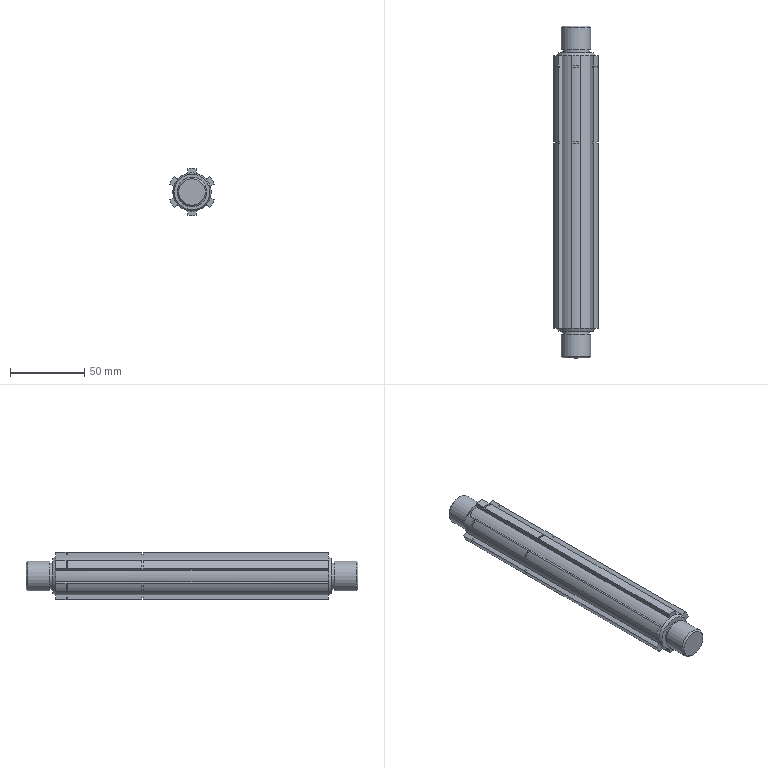Component | NX | ZHOU9 | 1 solid | 98 faces | volume 130612 mm3 | plane 54 | cylinder 40 | cone 4 | commonest cylinder face diameters 32 x18 30 x12 26 x6 18 x2 20 x2